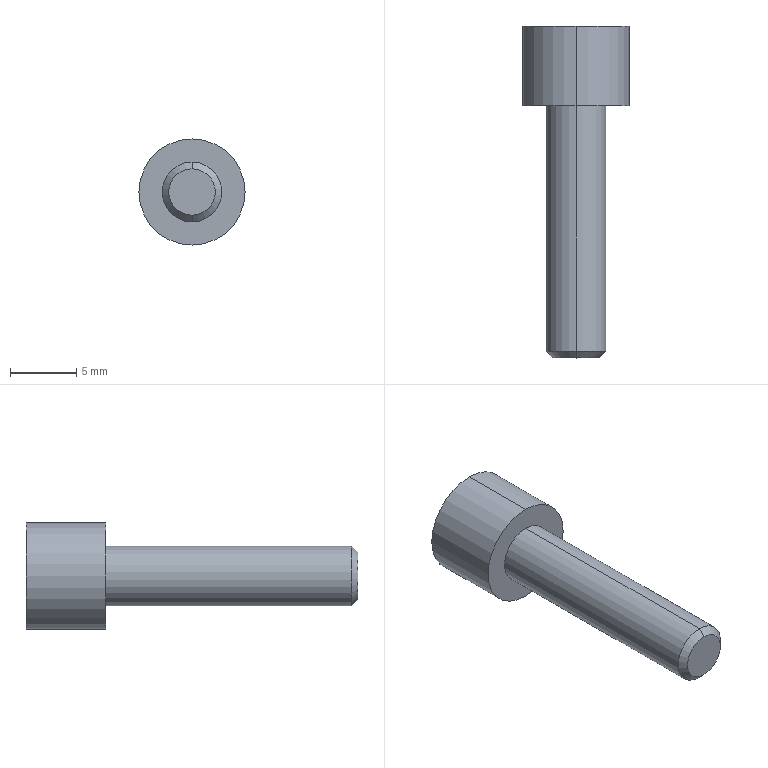Component | SolidWorks | CountersunkScrewM8x4-1 | 1 solid | 9 faces | box 8 x 25 x 8 mm | volume 602 mm3 | cylinder 4 | plane 3 | cone 2 | commonest cylinder face diameters 4.5 x2 8 x2
build123d program:
from build123d import *

# Parameters (mm, degrees)
SKETCH2_R           = 4
BOSS_EXTRUDE1_DEPTH = 10
SKETCH5_R           = 2.25
BOSS_EXTRUDE2_DEPTH = 29
CHAMFER1_SIZE       = 0.5
CUT_EXTRUDE1_DEPTH  = 4


with BuildPart() as part:
    # Sketch2 → Boss-Extrude1 (new body)
    with BuildSketch(Plane.XY.offset(20)):
        with Locations((20.473, -29.973)):
            Circle(SKETCH2_R)
    extrude(amount=-BOSS_EXTRUDE1_DEPTH)

    # Sketch5 → Boss-Extrude2 (add)
    with BuildSketch(Plane.XY.offset(20)):
        with Locations((20.473, -29.973)):
            Circle(SKETCH5_R)
    extrude(amount=-BOSS_EXTRUDE2_DEPTH)

    # Chamfer1
    chamfer1_edges = [part.edges().sort_by_distance(p)[0] for p in [
        (18.223, -29.973, -9),
    ]]
    chamfer(chamfer1_edges, length=CHAMFER1_SIZE)

    # Sketch6 → Cut-Extrude1 (cut)
    with BuildSketch(Plane.XY.offset(20)):
        Polygon((20.473, -8.425), (1.812, -19.199), (1.812, -40.747), (20.473, -51.521), (39.134, -40.747), (39.134, -19.199), align=None)
    extrude(amount=-CUT_EXTRUDE1_DEPTH, mode=Mode.SUBTRACT)


solid = part.part

# Placed as in the assembly
solid = solid.moved(Location((6.5, 96.74, -50.446), (-90, 0, 0)))
STEP:
#1=CARTESIAN_POINT('',(1.062,3.454,-0.7371));
#2=VERTEX_POINT('',#1);
#3=CARTESIAN_POINT('',(1.062,3.454,-0.8749));
#4=VERTEX_POINT('',#3);
#5=CARTESIAN_POINT('',(1.062,3.454,-0.806));
#6=DIRECTION('',(-0.,-1.,-0.));
#7=DIRECTION('',(0.,0.,-1.));
#8=AXIS2_PLACEMENT_3D('',#5,#6,#7);
#9=CIRCLE('',#8,0.0689);
#10=EDGE_CURVE('',#2,#4,#9,.T.);
#11=ORIENTED_EDGE('',*,*,#10,.F.);
#12=CARTESIAN_POINT('',(1.062,3.474,-0.7174));
#13=VERTEX_POINT('',#12);
#14=CARTESIAN_POINT('',(1.062,3.474,-0.7174));
#15=DIRECTION('',(-0.,0.7071,0.7071));
#16=VECTOR('',#15,39.37);
#17=LINE('',#14,#16);
#18=EDGE_CURVE('',#2,#13,#17,.T.);
#19=ORIENTED_EDGE('',*,*,#18,.T.);
#20=CARTESIAN_POINT('',(1.062,3.474,-0.8946));
#21=VERTEX_POINT('',#20);
#22=CARTESIAN_POINT('',(1.062,3.474,-0.806));
#23=DIRECTION('',(0.,1.,0.));
#24=DIRECTION('',(0.,0.,-1.));
#25=AXIS2_PLACEMENT_3D('',#22,#23,#24);
#26=CIRCLE('',#25,0.08858);
#27=EDGE_CURVE('',#21,#13,#26,.T.);
#28=ORIENTED_EDGE('',*,*,#27,.F.);
#29=CARTESIAN_POINT('',(1.062,3.474,-0.8946));
#30=DIRECTION('',(-0.,0.7071,-0.7071));
#31=VECTOR('',#30,39.37);
#32=LINE('',#29,#31);
#33=EDGE_CURVE('',#4,#21,#32,.T.);
#34=ORIENTED_EDGE('',*,*,#33,.F.);
#35=EDGE_LOOP('',(#11,#19,#28,#34));
#36=FACE_OUTER_BOUND('',#35,.T.);
#37=CARTESIAN_POINT('',(1.062,3.474,-0.806));
#38=DIRECTION('',(0.,1.,0.));
#39=DIRECTION('',(0.,0.,-1.));
#40=AXIS2_PLACEMENT_3D('',#37,#38,#39);
#41=CONICAL_SURFACE('',#40,0.08858,0.7854);
#42=ADVANCED_FACE('',(#36),#41,.T.);
#43=ORIENTED_EDGE('',*,*,#27,.T.);
#44=CARTESIAN_POINT('',(1.062,4.202,-0.7174));
#45=VERTEX_POINT('',#44);
#46=CARTESIAN_POINT('',(1.062,3.454,-0.7174));
#47=DIRECTION('',(0.,1.,0.));
#48=VECTOR('',#47,39.37);
#49=LINE('',#46,#48);
#50=EDGE_CURVE('',#13,#45,#49,.T.);
#51=ORIENTED_EDGE('',*,*,#50,.T.);
#52=CARTESIAN_POINT('',(1.062,4.202,-0.8946));
#53=VERTEX_POINT('',#52);
#54=CARTESIAN_POINT('',(1.062,4.202,-0.806));
#55=DIRECTION('',(0.,1.,-0.));
#56=DIRECTION('',(0.,0.,-1.));
#57=AXIS2_PLACEMENT_3D('',#54,#55,#56);
#58=CIRCLE('',#57,0.08858);
#59=EDGE_CURVE('',#53,#45,#58,.T.);
#60=ORIENTED_EDGE('',*,*,#59,.F.);
#61=CARTESIAN_POINT('',(1.062,3.454,-0.8946));
#62=DIRECTION('',(0.,1.,0.));
#63=VECTOR('',#62,39.37);
#64=LINE('',#61,#63);
#65=EDGE_CURVE('',#21,#53,#64,.T.);
#66=ORIENTED_EDGE('',*,*,#65,.F.);
#67=EDGE_LOOP('',(#43,#51,#60,#66));
#68=FACE_OUTER_BOUND('',#67,.T.);
#69=CARTESIAN_POINT('',(1.062,3.454,-0.806));
#70=DIRECTION('',(0.,1.,0.));
#71=DIRECTION('',(0.,0.,-1.));
#72=AXIS2_PLACEMENT_3D('',#69,#70,#71);
#73=CYLINDRICAL_SURFACE('',#72,0.08858);
#74=ADVANCED_FACE('',(#68),#73,.T.);
#75=CARTESIAN_POINT('',(1.062,4.202,-0.6485));
#76=VERTEX_POINT('',#75);
#77=CARTESIAN_POINT('',(1.062,4.202,-0.9635));
#78=VERTEX_POINT('',#77);
#79=CARTESIAN_POINT('',(1.062,4.202,-0.806));
#80=DIRECTION('',(-0.,-1.,0.));
#81=DIRECTION('',(0.,0.,-1.));
#82=AXIS2_PLACEMENT_3D('',#79,#80,#81);
#83=CIRCLE('',#82,0.1575);
#84=EDGE_CURVE('',#76,#78,#83,.T.);
#85=ORIENTED_EDGE('',*,*,#84,.F.);
#86=CARTESIAN_POINT('',(1.062,4.439,-0.6485));
#87=VERTEX_POINT('',#86);
#88=CARTESIAN_POINT('',(1.062,3.757,-0.6485));
#89=DIRECTION('',(0.,1.,0.));
#90=VECTOR('',#89,39.37);
#91=LINE('',#88,#90);
#92=EDGE_CURVE('',#76,#87,#91,.T.);
#93=ORIENTED_EDGE('',*,*,#92,.T.);
#94=CARTESIAN_POINT('',(1.062,4.439,-0.9635));
#95=VERTEX_POINT('',#94);
#96=CARTESIAN_POINT('',(1.062,4.439,-0.806));
#97=DIRECTION('',(-0.,-1.,-0.));
#98=DIRECTION('',(0.,0.,-1.));
#99=AXIS2_PLACEMENT_3D('',#96,#97,#98);
#100=CIRCLE('',#99,0.1575);
#101=EDGE_CURVE('',#87,#95,#100,.T.);
#102=ORIENTED_EDGE('',*,*,#101,.T.);
#103=CARTESIAN_POINT('',(1.062,3.757,-0.9635));
#104=DIRECTION('',(0.,1.,0.));
#105=VECTOR('',#104,39.37);
#106=LINE('',#103,#105);
#107=EDGE_CURVE('',#78,#95,#106,.T.);
#108=ORIENTED_EDGE('',*,*,#107,.F.);
#109=EDGE_LOOP('',(#85,#93,#102,#108));
#110=FACE_OUTER_BOUND('',#109,.T.);
#111=CARTESIAN_POINT('',(1.062,3.757,-0.806));
#112=DIRECTION('',(0.,1.,0.));
#113=DIRECTION('',(0.,0.,-1.));
#114=AXIS2_PLACEMENT_3D('',#111,#112,#113);
#115=CYLINDRICAL_SURFACE('',#114,0.1575);
#116=ADVANCED_FACE('',(#110),#115,.T.);
#117=ORIENTED_EDGE('',*,*,#92,.F.);
#118=CARTESIAN_POINT('',(1.062,4.202,-0.806));
#119=DIRECTION('',(-0.,-1.,0.));
#120=DIRECTION('',(0.,0.,-1.));
#121=AXIS2_PLACEMENT_3D('',#118,#119,#120);
#122=CIRCLE('',#121,0.1575);
#123=EDGE_CURVE('',#78,#76,#122,.T.);
#124=ORIENTED_EDGE('',*,*,#123,.F.);
#125=ORIENTED_EDGE('',*,*,#107,.T.);
#126=CARTESIAN_POINT('',(1.062,4.439,-0.806));
#127=DIRECTION('',(-0.,-1.,-0.));
#128=DIRECTION('',(0.,0.,-1.));
#129=AXIS2_PLACEMENT_3D('',#126,#127,#128);
#130=CIRCLE('',#129,0.1575);
#131=EDGE_CURVE('',#95,#87,#130,.T.);
#132=ORIENTED_EDGE('',*,*,#131,.T.);
#133=EDGE_LOOP('',(#117,#124,#125,#132));
#134=FACE_OUTER_BOUND('',#133,.T.);
#135=CARTESIAN_POINT('',(1.062,3.757,-0.806));
#136=DIRECTION('',(0.,1.,0.));
#137=DIRECTION('',(0.,0.,-1.));
#138=AXIS2_PLACEMENT_3D('',#135,#136,#137);
#139=CYLINDRICAL_SURFACE('',#138,0.1575);
#140=ADVANCED_FACE('',(#134),#139,.T.);
#141=ORIENTED_EDGE('',*,*,#59,.T.);
#142=CARTESIAN_POINT('',(1.062,4.202,-0.806));
#143=DIRECTION('',(0.,1.,-0.));
#144=DIRECTION('',(0.,0.,-1.));
#145=AXIS2_PLACEMENT_3D('',#142,#143,#144);
#146=CIRCLE('',#145,0.08858);
#147=EDGE_CURVE('',#45,#53,#146,.T.);
#148=ORIENTED_EDGE('',*,*,#147,.T.);
#149=EDGE_LOOP('',(#141,#148));
#150=FACE_BOUND('',#149,.T.);
#151=ORIENTED_EDGE('',*,*,#123,.T.);
#152=ORIENTED_EDGE('',*,*,#84,.T.);
#153=EDGE_LOOP('',(#151,#152));
#154=FACE_OUTER_BOUND('',#153,.T.);
#155=CARTESIAN_POINT('',(1.062,4.202,-0.806));
#156=DIRECTION('',(0.,1.,-0.));
#157=DIRECTION('',(1.,-0.,-0.));
#158=AXIS2_PLACEMENT_3D('',#155,#156,#157);
#159=PLANE('',#158);
#160=ADVANCED_FACE('',(#150,#154),#159,.F.);
#161=ORIENTED_EDGE('',*,*,#50,.F.);
#162=CARTESIAN_POINT('',(1.062,3.474,-0.806));
#163=DIRECTION('',(0.,1.,0.));
#164=DIRECTION('',(0.,0.,-1.));
#165=AXIS2_PLACEMENT_3D('',#162,#163,#164);
#166=CIRCLE('',#165,0.08858);
#167=EDGE_CURVE('',#13,#21,#166,.T.);
#168=ORIENTED_EDGE('',*,*,#167,.T.);
#169=ORIENTED_EDGE('',*,*,#65,.T.);
#170=ORIENTED_EDGE('',*,*,#147,.F.);
#171=EDGE_LOOP('',(#161,#168,#169,#170));
#172=FACE_OUTER_BOUND('',#171,.T.);
#173=CARTESIAN_POINT('',(1.062,3.454,-0.806));
#174=DIRECTION('',(0.,1.,0.));
#175=DIRECTION('',(0.,0.,-1.));
#176=AXIS2_PLACEMENT_3D('',#173,#174,#175);
#177=CYLINDRICAL_SURFACE('',#176,0.08858);
#178=ADVANCED_FACE('',(#172),#177,.T.);
#179=CARTESIAN_POINT('',(1.062,3.454,-0.806));
#180=DIRECTION('',(-0.,-1.,-0.));
#181=DIRECTION('',(0.,0.,-1.));
#182=AXIS2_PLACEMENT_3D('',#179,#180,#181);
#183=CIRCLE('',#182,0.0689);
#184=EDGE_CURVE('',#4,#2,#183,.T.);
#185=ORIENTED_EDGE('',*,*,#184,.T.);
#186=ORIENTED_EDGE('',*,*,#10,.T.);
#187=EDGE_LOOP('',(#185,#186));
#188=FACE_OUTER_BOUND('',#187,.T.);
#189=CARTESIAN_POINT('',(1.062,3.454,-0.806));
#190=DIRECTION('',(0.,1.,0.));
#191=DIRECTION('',(-0.,0.,-1.));
#192=AXIS2_PLACEMENT_3D('',#189,#190,#191);
#193=PLANE('',#192);
#194=ADVANCED_FACE('',(#188),#193,.F.);
#195=ORIENTED_EDGE('',*,*,#18,.F.);
#196=ORIENTED_EDGE('',*,*,#184,.F.);
#197=ORIENTED_EDGE('',*,*,#33,.T.);
#198=ORIENTED_EDGE('',*,*,#167,.F.);
#199=EDGE_LOOP('',(#195,#196,#197,#198));
#200=FACE_OUTER_BOUND('',#199,.T.);
#201=CARTESIAN_POINT('',(1.062,3.474,-0.806));
#202=DIRECTION('',(0.,1.,0.));
#203=DIRECTION('',(0.,0.,-1.));
#204=AXIS2_PLACEMENT_3D('',#201,#202,#203);
#205=CONICAL_SURFACE('',#204,0.08858,0.7854);
#206=ADVANCED_FACE('',(#200),#205,.T.);
#207=ORIENTED_EDGE('',*,*,#131,.F.);
#208=ORIENTED_EDGE('',*,*,#101,.F.);
#209=EDGE_LOOP('',(#207,#208));
#210=FACE_OUTER_BOUND('',#209,.T.);
#211=CARTESIAN_POINT('',(-0.1181,4.439,-0.));
#212=DIRECTION('',(0.,1.,0.));
#213=DIRECTION('',(-0.,0.,-1.));
#214=AXIS2_PLACEMENT_3D('',#211,#212,#213);
#215=PLANE('',#214);
#216=ADVANCED_FACE('',(#210),#215,.T.);
#217=CLOSED_SHELL('',(#42,#74,#116,#140,#160,#178,#194,#206,#216));
#218=MANIFOLD_SOLID_BREP('',#217);
#219=CARTESIAN_POINT('',(0.,0.,0.));
#220=DIRECTION('',(0.,0.,1.));
#221=DIRECTION('',(1.,0.,0.));
#222=AXIS2_PLACEMENT_3D('',#219,#220,#221);
#223=(LENGTH_UNIT()NAMED_UNIT(*)SI_UNIT($,.METRE.));
#224=LENGTH_MEASURE_WITH_UNIT(LENGTH_MEASURE(0.0254),#223);
#225=DIMENSIONAL_EXPONENTS(1.,0.,0.,0.,0.,0.,0.);
#226=(CONVERSION_BASED_UNIT('',#224)LENGTH_UNIT()NAMED_UNIT(#225));
#227=UNCERTAINTY_MEASURE_WITH_UNIT(LENGTH_MEASURE(0.00001),#226,'','');
#228=(NAMED_UNIT(*)PLANE_ANGLE_UNIT()SI_UNIT($,.RADIAN.));
#229=(NAMED_UNIT(*)SI_UNIT($,.STERADIAN.)SOLID_ANGLE_UNIT());
#230=(GEOMETRIC_REPRESENTATION_CONTEXT(3)GLOBAL_UNCERTAINTY_ASSIGNED_CONTEXT((#227))GLOBAL_UNIT_ASSIGNED_CONTEXT((#226,#228,#229))REPRESENTATION_CONTEXT('',''));
#231=ADVANCED_BREP_SHAPE_REPRESENTATION('',(#218,#222),#230);
#232=COLOUR_RGB('',0.7922,0.8196,0.9333);
#233=FILL_AREA_STYLE_COLOUR('',#232);
#234=FILL_AREA_STYLE('',(#233));
#235=SURFACE_STYLE_FILL_AREA(#234);
#236=SURFACE_SIDE_STYLE('',(#235));
#237=SURFACE_STYLE_USAGE(.BOTH.,#236);
#238=PRESENTATION_STYLE_ASSIGNMENT((#237));
#239=STYLED_ITEM('',(#238),#218);
#240=(LENGTH_UNIT()NAMED_UNIT(*)SI_UNIT($,.METRE.));
#241=LENGTH_MEASURE_WITH_UNIT(LENGTH_MEASURE(0.0254),#240);
#242=DIMENSIONAL_EXPONENTS(1.,0.,0.,0.,0.,0.,0.);
#243=(CONVERSION_BASED_UNIT('',#241)LENGTH_UNIT()NAMED_UNIT(#242));
#244=UNCERTAINTY_MEASURE_WITH_UNIT(LENGTH_MEASURE(0.00001),#243,'','');
#245=(NAMED_UNIT(*)PLANE_ANGLE_UNIT()SI_UNIT($,.RADIAN.));
#246=(NAMED_UNIT(*)SI_UNIT($,.STERADIAN.)SOLID_ANGLE_UNIT());
#247=(GEOMETRIC_REPRESENTATION_CONTEXT(3)GLOBAL_UNCERTAINTY_ASSIGNED_CONTEXT((#244))GLOBAL_UNIT_ASSIGNED_CONTEXT((#243,#245,#246))REPRESENTATION_CONTEXT('',''));
#248=MECHANICAL_DESIGN_GEOMETRIC_PRESENTATION_REPRESENTATION('',(#239),#247);
#249=PRESENTATION_LAYER_ASSIGNMENT('','',(#239));